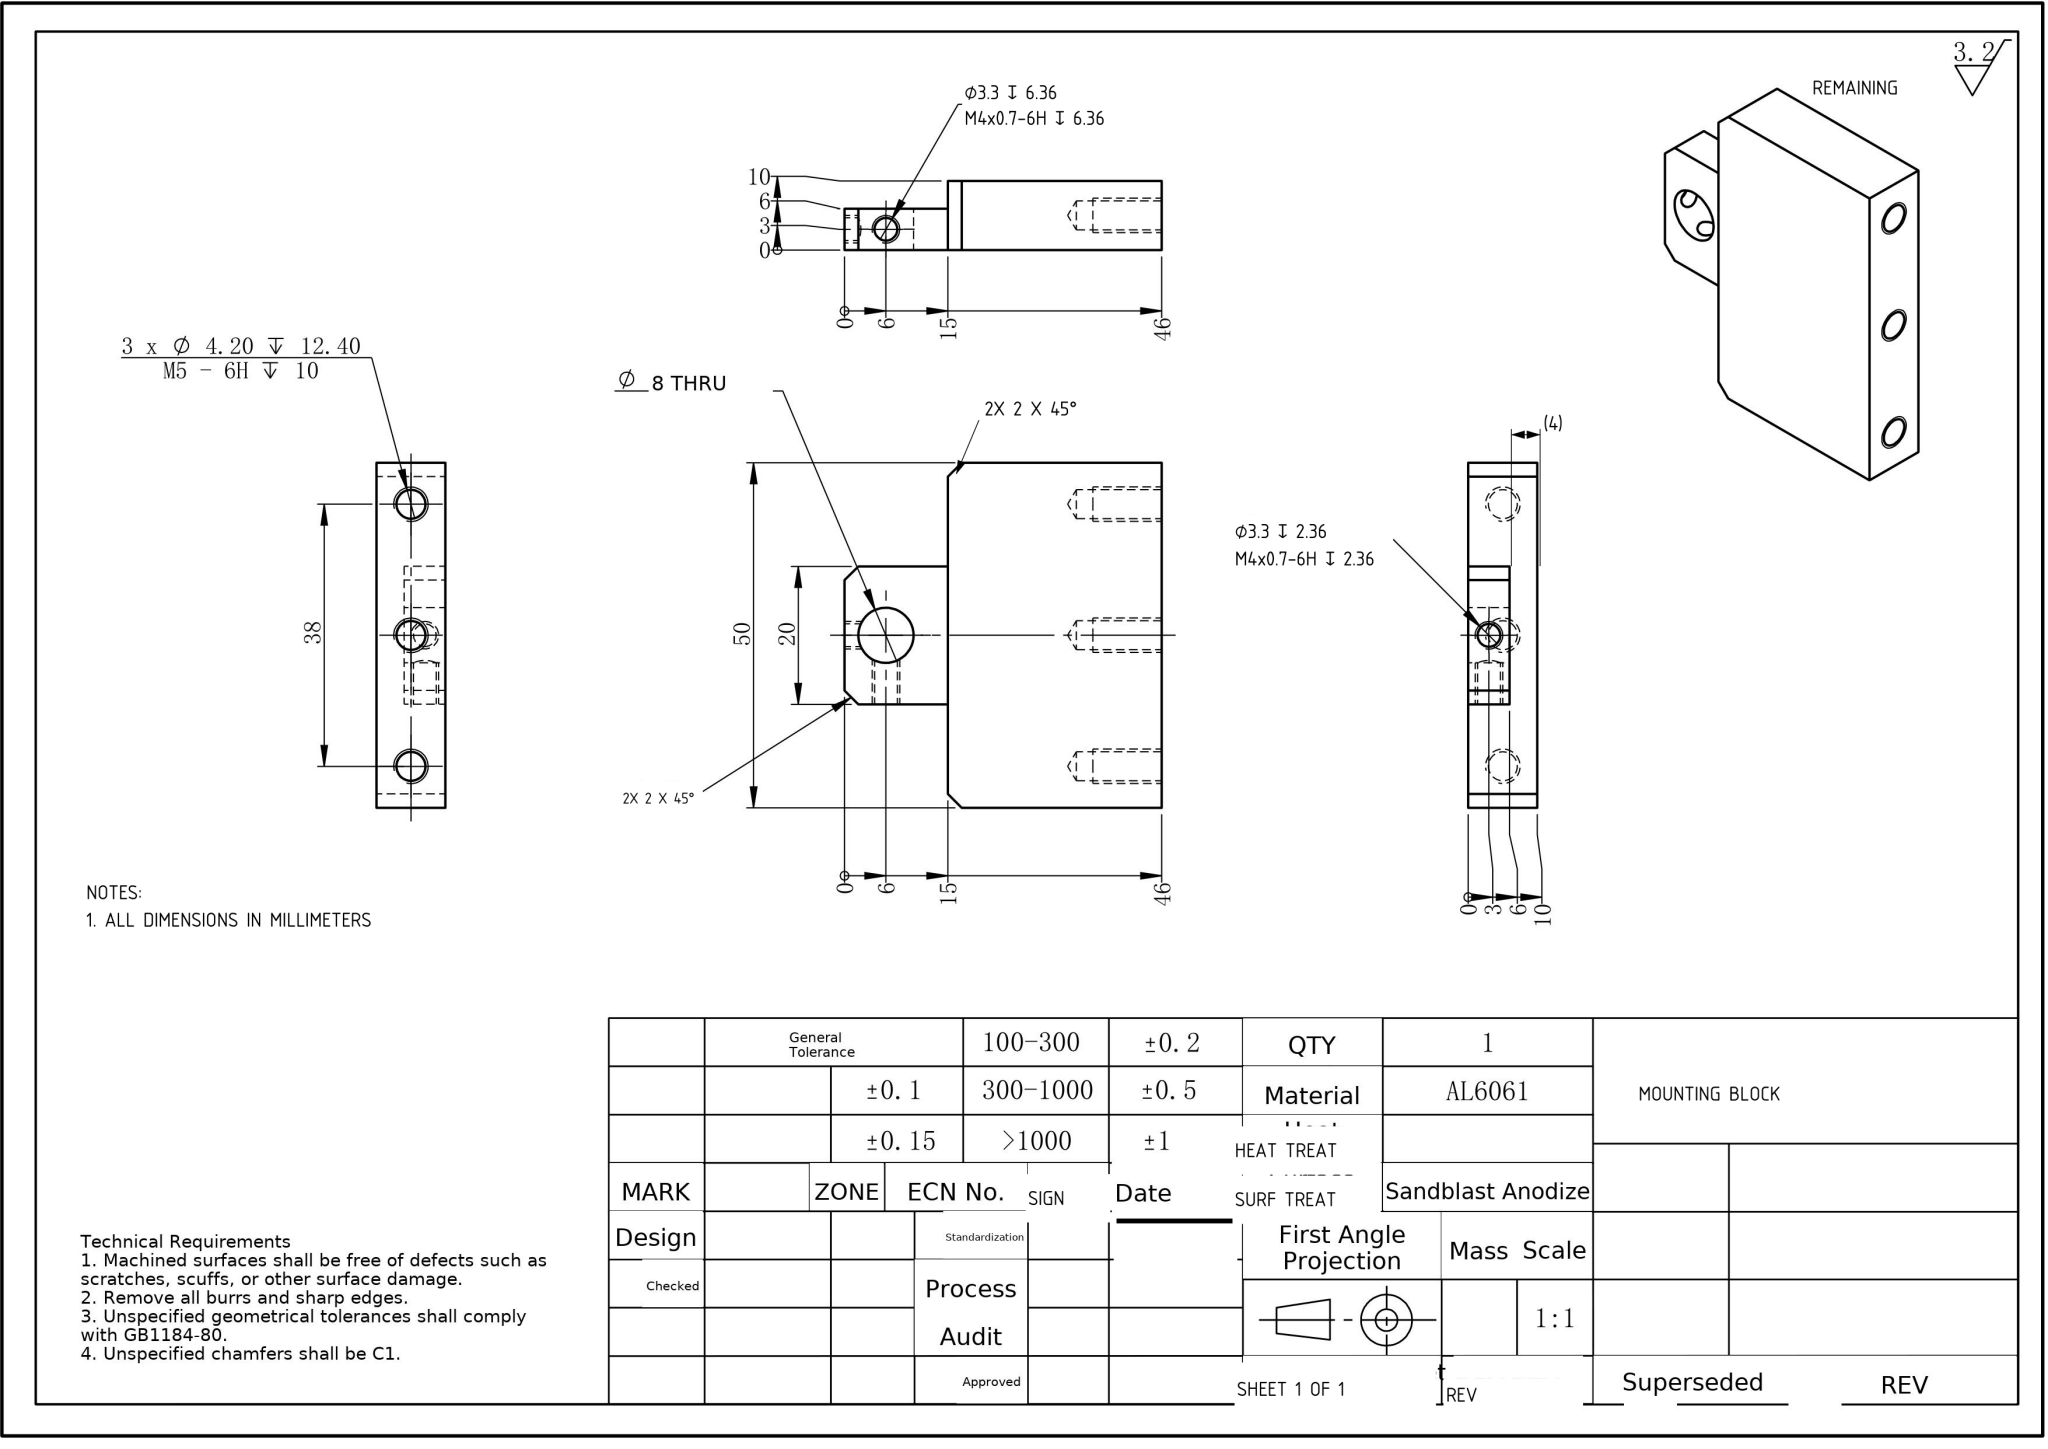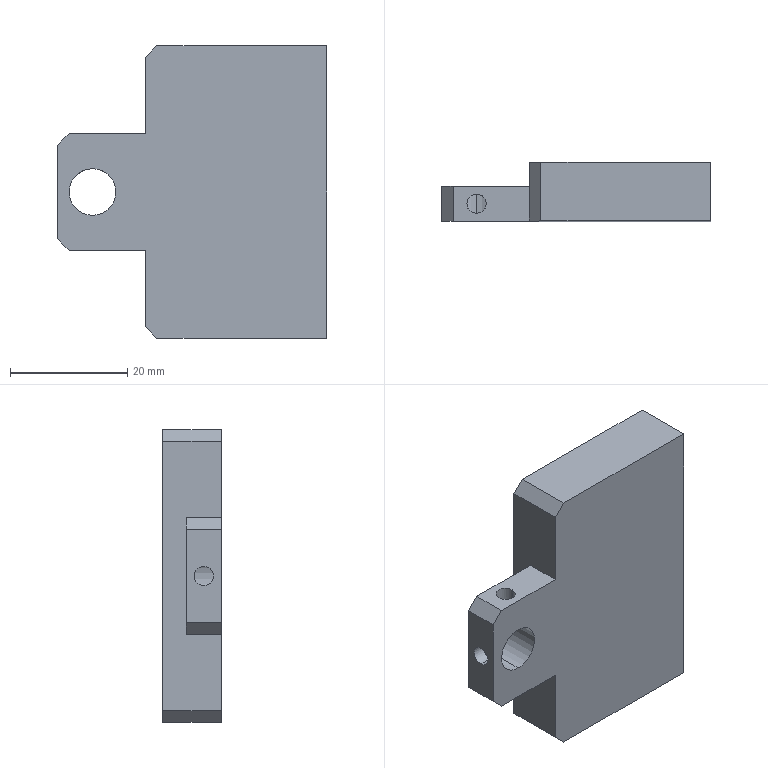Part | NX | mm | 1 solid | 32 faces | box 46 x 10 x 50 mm | volume 16332 mm3 | plane 14 | cylinder 12 | cone 6 | commonest cylinder face diameters 4.2 x6 3.3 x4 8 x2